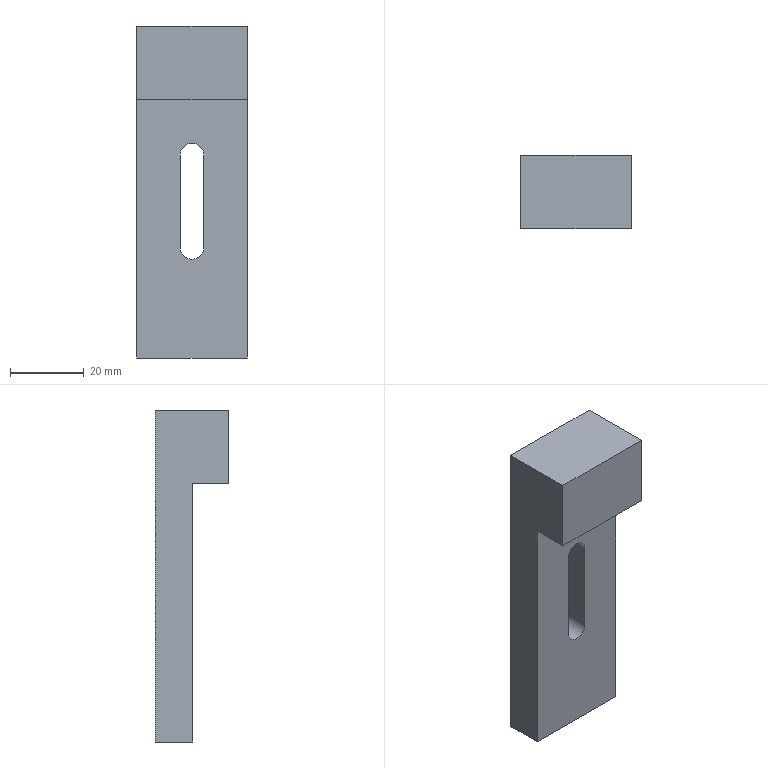Component | SolidWorks | CS021-A10-A012-3 | 1 solid | 12 faces | box 30 x 20 x 90 mm | volume 31424 mm3 | plane 10 | cylinder 2 | commonest cylinder face diameters 6.5 x2 | material AL6061
build123d program:
from build123d import *

# Parameters (mm, degrees)
BOSS_EXTRUDE1_DEPTH = 15
CUT_EXTRUDE1_REACH  = 95.408


with BuildPart() as part:
    # Sketch1 → Boss-Extrude1 (new, symmetric)
    with BuildSketch(Plane.XY):
        Polygon((0, 0), (0, 20), (90, 20), (90, 9.8), (20, 9.8), (20, 0), align=None)
    extrude(amount=BOSS_EXTRUDE1_DEPTH, both=True)

    # Sketch2 → Cut-Extrude1 (cut, up to next)
    with BuildSketch(Plane(origin=(0, 20, 0), x_dir=(1, 0, 0), z_dir=(0, 1, 0)), mode=Mode.PRIVATE) as cut_extrude1_sk1:
        with BuildLine():
            Line((35, 3.25), (60, 3.25))
            ThreePointArc((60, 3.25), (63.25, 0), (60, -3.25))
            Line((60, -3.25), (35, -3.25))
            ThreePointArc((35, -3.25), (31.75, 0), (35, 3.25))
        make_face()
    cut_extrude1_tool1 = extrude(cut_extrude1_sk1.sketch, amount=-CUT_EXTRUDE1_REACH, mode=Mode.PRIVATE) & part.part
    add(cut_extrude1_tool1.solids().sort_by_distance((47.5, 20, 0))[0], mode=Mode.SUBTRACT)


solid = part.part

# Placed as in the assembly
solid = solid.moved(Location((197.949, 15.017, 130), (0, 90, 0)))
STEP:
#1=COLOUR_RGB('',0.7922,0.8196,0.9333);
#2=FILL_AREA_STYLE_COLOUR('',#1);
#3=FILL_AREA_STYLE('',(#2));
#4=SURFACE_STYLE_FILL_AREA(#3);
#5=SURFACE_SIDE_STYLE('',(#4));
#6=SURFACE_STYLE_USAGE(.BOTH.,#5);
#7=PRESENTATION_STYLE_ASSIGNMENT((#6));
#8=CARTESIAN_POINT('',(7.203,0.5912,5.118));
#9=VERTEX_POINT('',#8);
#10=CARTESIAN_POINT('',(7.203,0.5912,4.331));
#11=VERTEX_POINT('',#10);
#12=CARTESIAN_POINT('',(7.203,0.5912,4.331));
#13=DIRECTION('',(0.,-0.,-1.));
#14=VECTOR('',#13,39.37);
#15=LINE('',#12,#14);
#16=EDGE_CURVE('',#9,#11,#15,.T.);
#17=ORIENTED_EDGE('',*,*,#16,.T.);
#18=CARTESIAN_POINT('',(8.384,0.5912,4.331));
#19=VERTEX_POINT('',#18);
#20=CARTESIAN_POINT('',(8.384,0.5912,4.331));
#21=DIRECTION('',(-1.,0.,0.));
#22=VECTOR('',#21,39.37);
#23=LINE('',#20,#22);
#24=EDGE_CURVE('',#19,#11,#23,.T.);
#25=ORIENTED_EDGE('',*,*,#24,.F.);
#26=CARTESIAN_POINT('',(8.384,0.5912,5.118));
#27=VERTEX_POINT('',#26);
#28=CARTESIAN_POINT('',(8.384,0.5912,4.331));
#29=DIRECTION('',(0.,-0.,-1.));
#30=VECTOR('',#29,39.37);
#31=LINE('',#28,#30);
#32=EDGE_CURVE('',#27,#19,#31,.T.);
#33=ORIENTED_EDGE('',*,*,#32,.F.);
#34=CARTESIAN_POINT('',(8.384,0.5912,5.118));
#35=DIRECTION('',(-1.,0.,0.));
#36=VECTOR('',#35,39.37);
#37=LINE('',#34,#36);
#38=EDGE_CURVE('',#27,#9,#37,.T.);
#39=ORIENTED_EDGE('',*,*,#38,.T.);
#40=EDGE_LOOP('',(#17,#25,#33,#39));
#41=FACE_OUTER_BOUND('',#40,.T.);
#42=CARTESIAN_POINT('',(8.384,0.5912,4.331));
#43=DIRECTION('',(0.,1.,-0.));
#44=DIRECTION('',(1.,-0.,0.));
#45=AXIS2_PLACEMENT_3D('',#42,#43,#44);
#46=PLANE('',#45);
#47=ADVANCED_FACE('',(#41),#46,.F.);
#48=CARTESIAN_POINT('',(7.203,0.977,4.331));
#49=VERTEX_POINT('',#48);
#50=CARTESIAN_POINT('',(7.203,0.977,4.331));
#51=DIRECTION('',(0.,1.,-0.));
#52=VECTOR('',#51,39.37);
#53=LINE('',#50,#52);
#54=EDGE_CURVE('',#11,#49,#53,.T.);
#55=ORIENTED_EDGE('',*,*,#54,.T.);
#56=CARTESIAN_POINT('',(8.384,0.977,4.331));
#57=VERTEX_POINT('',#56);
#58=CARTESIAN_POINT('',(8.384,0.977,4.331));
#59=DIRECTION('',(-1.,0.,0.));
#60=VECTOR('',#59,39.37);
#61=LINE('',#58,#60);
#62=EDGE_CURVE('',#57,#49,#61,.T.);
#63=ORIENTED_EDGE('',*,*,#62,.F.);
#64=CARTESIAN_POINT('',(8.384,0.977,4.331));
#65=DIRECTION('',(0.,1.,-0.));
#66=VECTOR('',#65,39.37);
#67=LINE('',#64,#66);
#68=EDGE_CURVE('',#19,#57,#67,.T.);
#69=ORIENTED_EDGE('',*,*,#68,.F.);
#70=ORIENTED_EDGE('',*,*,#24,.T.);
#71=EDGE_LOOP('',(#55,#63,#69,#70));
#72=FACE_OUTER_BOUND('',#71,.T.);
#73=CARTESIAN_POINT('',(8.384,0.977,4.331));
#74=DIRECTION('',(-0.,0.,1.));
#75=DIRECTION('',(-0.,-1.,0.));
#76=AXIS2_PLACEMENT_3D('',#73,#74,#75);
#77=PLANE('',#76);
#78=ADVANCED_FACE('',(#72),#77,.F.);
#79=CARTESIAN_POINT('',(7.665,0.977,3.74));
#80=VERTEX_POINT('',#79);
#81=CARTESIAN_POINT('',(7.665,0.977,2.756));
#82=VERTEX_POINT('',#81);
#83=CARTESIAN_POINT('',(7.665,0.977,3.74));
#84=DIRECTION('',(0.,0.,-1.));
#85=VECTOR('',#84,39.37);
#86=LINE('',#83,#85);
#87=EDGE_CURVE('',#80,#82,#86,.T.);
#88=ORIENTED_EDGE('',*,*,#87,.F.);
#89=CARTESIAN_POINT('',(7.921,0.977,3.74));
#90=VERTEX_POINT('',#89);
#91=CARTESIAN_POINT('',(7.793,0.977,3.74));
#92=DIRECTION('',(-0.,-1.,-0.));
#93=DIRECTION('',(0.,0.,1.));
#94=AXIS2_PLACEMENT_3D('',#91,#92,#93);
#95=CIRCLE('',#94,0.128);
#96=EDGE_CURVE('',#90,#80,#95,.T.);
#97=ORIENTED_EDGE('',*,*,#96,.F.);
#98=CARTESIAN_POINT('',(7.921,0.977,2.756));
#99=VERTEX_POINT('',#98);
#100=CARTESIAN_POINT('',(7.921,0.977,3.74));
#101=DIRECTION('',(-0.,-0.,1.));
#102=VECTOR('',#101,39.37);
#103=LINE('',#100,#102);
#104=EDGE_CURVE('',#99,#90,#103,.T.);
#105=ORIENTED_EDGE('',*,*,#104,.F.);
#106=CARTESIAN_POINT('',(7.793,0.977,2.756));
#107=DIRECTION('',(-0.,-1.,-0.));
#108=DIRECTION('',(0.,0.,1.));
#109=AXIS2_PLACEMENT_3D('',#106,#107,#108);
#110=CIRCLE('',#109,0.128);
#111=EDGE_CURVE('',#82,#99,#110,.T.);
#112=ORIENTED_EDGE('',*,*,#111,.F.);
#113=EDGE_LOOP('',(#88,#97,#105,#112));
#114=FACE_BOUND('',#113,.T.);
#115=CARTESIAN_POINT('',(7.203,0.977,1.575));
#116=VERTEX_POINT('',#115);
#117=CARTESIAN_POINT('',(7.203,0.977,1.575));
#118=DIRECTION('',(0.,0.,-1.));
#119=VECTOR('',#118,39.37);
#120=LINE('',#117,#119);
#121=EDGE_CURVE('',#49,#116,#120,.T.);
#122=ORIENTED_EDGE('',*,*,#121,.T.);
#123=CARTESIAN_POINT('',(8.384,0.977,1.575));
#124=VERTEX_POINT('',#123);
#125=CARTESIAN_POINT('',(8.384,0.977,1.575));
#126=DIRECTION('',(-1.,0.,0.));
#127=VECTOR('',#126,39.37);
#128=LINE('',#125,#127);
#129=EDGE_CURVE('',#124,#116,#128,.T.);
#130=ORIENTED_EDGE('',*,*,#129,.F.);
#131=CARTESIAN_POINT('',(8.384,0.977,1.575));
#132=DIRECTION('',(0.,0.,-1.));
#133=VECTOR('',#132,39.37);
#134=LINE('',#131,#133);
#135=EDGE_CURVE('',#57,#124,#134,.T.);
#136=ORIENTED_EDGE('',*,*,#135,.F.);
#137=ORIENTED_EDGE('',*,*,#62,.T.);
#138=EDGE_LOOP('',(#122,#130,#136,#137));
#139=FACE_OUTER_BOUND('',#138,.T.);
#140=CARTESIAN_POINT('',(8.384,0.977,1.575));
#141=DIRECTION('',(0.,1.,0.));
#142=DIRECTION('',(-0.,-0.,1.));
#143=AXIS2_PLACEMENT_3D('',#140,#141,#142);
#144=PLANE('',#143);
#145=ADVANCED_FACE('',(#114,#139),#144,.F.);
#146=CARTESIAN_POINT('',(7.203,1.379,1.575));
#147=VERTEX_POINT('',#146);
#148=CARTESIAN_POINT('',(7.203,1.379,1.575));
#149=DIRECTION('',(0.,1.,-0.));
#150=VECTOR('',#149,39.37);
#151=LINE('',#148,#150);
#152=EDGE_CURVE('',#116,#147,#151,.T.);
#153=ORIENTED_EDGE('',*,*,#152,.T.);
#154=CARTESIAN_POINT('',(8.384,1.379,1.575));
#155=VERTEX_POINT('',#154);
#156=CARTESIAN_POINT('',(8.384,1.379,1.575));
#157=DIRECTION('',(-1.,0.,0.));
#158=VECTOR('',#157,39.37);
#159=LINE('',#156,#158);
#160=EDGE_CURVE('',#155,#147,#159,.T.);
#161=ORIENTED_EDGE('',*,*,#160,.F.);
#162=CARTESIAN_POINT('',(8.384,1.379,1.575));
#163=DIRECTION('',(0.,1.,-0.));
#164=VECTOR('',#163,39.37);
#165=LINE('',#162,#164);
#166=EDGE_CURVE('',#124,#155,#165,.T.);
#167=ORIENTED_EDGE('',*,*,#166,.F.);
#168=ORIENTED_EDGE('',*,*,#129,.T.);
#169=EDGE_LOOP('',(#153,#161,#167,#168));
#170=FACE_OUTER_BOUND('',#169,.T.);
#171=CARTESIAN_POINT('',(8.384,1.379,1.575));
#172=DIRECTION('',(0.,0.,1.));
#173=DIRECTION('',(1.,-0.,0.));
#174=AXIS2_PLACEMENT_3D('',#171,#172,#173);
#175=PLANE('',#174);
#176=ADVANCED_FACE('',(#170),#175,.F.);
#177=CARTESIAN_POINT('',(7.921,1.379,3.74));
#178=VERTEX_POINT('',#177);
#179=CARTESIAN_POINT('',(7.921,1.379,2.756));
#180=VERTEX_POINT('',#179);
#181=CARTESIAN_POINT('',(7.921,1.379,3.74));
#182=DIRECTION('',(0.,-0.,-1.));
#183=VECTOR('',#182,39.37);
#184=LINE('',#181,#183);
#185=EDGE_CURVE('',#178,#180,#184,.T.);
#186=ORIENTED_EDGE('',*,*,#185,.F.);
#187=CARTESIAN_POINT('',(7.665,1.379,3.74));
#188=VERTEX_POINT('',#187);
#189=CARTESIAN_POINT('',(7.793,1.379,3.74));
#190=DIRECTION('',(0.,1.,-0.));
#191=DIRECTION('',(1.,0.,0.));
#192=AXIS2_PLACEMENT_3D('',#189,#190,#191);
#193=CIRCLE('',#192,0.128);
#194=EDGE_CURVE('',#188,#178,#193,.T.);
#195=ORIENTED_EDGE('',*,*,#194,.F.);
#196=CARTESIAN_POINT('',(7.665,1.379,2.756));
#197=VERTEX_POINT('',#196);
#198=CARTESIAN_POINT('',(7.665,1.379,3.74));
#199=DIRECTION('',(-0.,0.,1.));
#200=VECTOR('',#199,39.37);
#201=LINE('',#198,#200);
#202=EDGE_CURVE('',#197,#188,#201,.T.);
#203=ORIENTED_EDGE('',*,*,#202,.F.);
#204=CARTESIAN_POINT('',(7.793,1.379,2.756));
#205=DIRECTION('',(0.,1.,-0.));
#206=DIRECTION('',(1.,0.,0.));
#207=AXIS2_PLACEMENT_3D('',#204,#205,#206);
#208=CIRCLE('',#207,0.128);
#209=EDGE_CURVE('',#180,#197,#208,.T.);
#210=ORIENTED_EDGE('',*,*,#209,.F.);
#211=EDGE_LOOP('',(#186,#195,#203,#210));
#212=FACE_BOUND('',#211,.T.);
#213=CARTESIAN_POINT('',(7.203,1.379,5.118));
#214=VERTEX_POINT('',#213);
#215=CARTESIAN_POINT('',(7.203,1.379,5.118));
#216=DIRECTION('',(-0.,0.,1.));
#217=VECTOR('',#216,39.37);
#218=LINE('',#215,#217);
#219=EDGE_CURVE('',#147,#214,#218,.T.);
#220=ORIENTED_EDGE('',*,*,#219,.T.);
#221=CARTESIAN_POINT('',(8.384,1.379,5.118));
#222=VERTEX_POINT('',#221);
#223=CARTESIAN_POINT('',(8.384,1.379,5.118));
#224=DIRECTION('',(-1.,0.,0.));
#225=VECTOR('',#224,39.37);
#226=LINE('',#223,#225);
#227=EDGE_CURVE('',#222,#214,#226,.T.);
#228=ORIENTED_EDGE('',*,*,#227,.F.);
#229=CARTESIAN_POINT('',(8.384,1.379,5.118));
#230=DIRECTION('',(-0.,0.,1.));
#231=VECTOR('',#230,39.37);
#232=LINE('',#229,#231);
#233=EDGE_CURVE('',#155,#222,#232,.T.);
#234=ORIENTED_EDGE('',*,*,#233,.F.);
#235=ORIENTED_EDGE('',*,*,#160,.T.);
#236=EDGE_LOOP('',(#220,#228,#234,#235));
#237=FACE_OUTER_BOUND('',#236,.T.);
#238=CARTESIAN_POINT('',(8.384,1.379,5.118));
#239=DIRECTION('',(-0.,-1.,0.));
#240=DIRECTION('',(-1.,0.,0.));
#241=AXIS2_PLACEMENT_3D('',#238,#239,#240);
#242=PLANE('',#241);
#243=ADVANCED_FACE('',(#212,#237),#242,.F.);
#244=CARTESIAN_POINT('',(7.203,0.5912,5.118));
#245=DIRECTION('',(-0.,-1.,0.));
#246=VECTOR('',#245,39.37);
#247=LINE('',#244,#246);
#248=EDGE_CURVE('',#214,#9,#247,.T.);
#249=ORIENTED_EDGE('',*,*,#248,.T.);
#250=ORIENTED_EDGE('',*,*,#38,.F.);
#251=CARTESIAN_POINT('',(8.384,0.5912,5.118));
#252=DIRECTION('',(-0.,-1.,0.));
#253=VECTOR('',#252,39.37);
#254=LINE('',#251,#253);
#255=EDGE_CURVE('',#222,#27,#254,.T.);
#256=ORIENTED_EDGE('',*,*,#255,.F.);
#257=ORIENTED_EDGE('',*,*,#227,.T.);
#258=EDGE_LOOP('',(#249,#250,#256,#257));
#259=FACE_OUTER_BOUND('',#258,.T.);
#260=CARTESIAN_POINT('',(8.384,0.5912,5.118));
#261=DIRECTION('',(-0.,-0.,-1.));
#262=DIRECTION('',(-1.,0.,0.));
#263=AXIS2_PLACEMENT_3D('',#260,#261,#262);
#264=PLANE('',#263);
#265=ADVANCED_FACE('',(#259),#264,.F.);
#266=ORIENTED_EDGE('',*,*,#32,.T.);
#267=ORIENTED_EDGE('',*,*,#68,.T.);
#268=ORIENTED_EDGE('',*,*,#135,.T.);
#269=ORIENTED_EDGE('',*,*,#166,.T.);
#270=ORIENTED_EDGE('',*,*,#233,.T.);
#271=ORIENTED_EDGE('',*,*,#255,.T.);
#272=EDGE_LOOP('',(#266,#267,#268,#269,#270,#271));
#273=FACE_OUTER_BOUND('',#272,.T.);
#274=CARTESIAN_POINT('',(8.384,0.5912,5.118));
#275=DIRECTION('',(-1.,0.,-0.));
#276=DIRECTION('',(-0.,0.,1.));
#277=AXIS2_PLACEMENT_3D('',#274,#275,#276);
#278=PLANE('',#277);
#279=ADVANCED_FACE('',(#273),#278,.F.);
#280=ORIENTED_EDGE('',*,*,#16,.F.);
#281=ORIENTED_EDGE('',*,*,#248,.F.);
#282=ORIENTED_EDGE('',*,*,#219,.F.);
#283=ORIENTED_EDGE('',*,*,#152,.F.);
#284=ORIENTED_EDGE('',*,*,#121,.F.);
#285=ORIENTED_EDGE('',*,*,#54,.F.);
#286=EDGE_LOOP('',(#280,#281,#282,#283,#284,#285));
#287=FACE_OUTER_BOUND('',#286,.T.);
#288=CARTESIAN_POINT('',(7.203,0.5912,5.118));
#289=DIRECTION('',(-1.,0.,-0.));
#290=DIRECTION('',(-0.,0.,1.));
#291=AXIS2_PLACEMENT_3D('',#288,#289,#290);
#292=PLANE('',#291);
#293=ADVANCED_FACE('',(#287),#292,.T.);
#294=ORIENTED_EDGE('',*,*,#96,.T.);
#295=CARTESIAN_POINT('',(7.665,0.5912,3.74));
#296=DIRECTION('',(0.,1.,-0.));
#297=VECTOR('',#296,39.37);
#298=LINE('',#295,#297);
#299=EDGE_CURVE('',#80,#188,#298,.T.);
#300=ORIENTED_EDGE('',*,*,#299,.T.);
#301=ORIENTED_EDGE('',*,*,#194,.T.);
#302=CARTESIAN_POINT('',(7.921,0.5912,3.74));
#303=DIRECTION('',(0.,1.,-0.));
#304=VECTOR('',#303,39.37);
#305=LINE('',#302,#304);
#306=EDGE_CURVE('',#90,#178,#305,.T.);
#307=ORIENTED_EDGE('',*,*,#306,.F.);
#308=EDGE_LOOP('',(#294,#300,#301,#307));
#309=FACE_OUTER_BOUND('',#308,.T.);
#310=CARTESIAN_POINT('',(7.793,0.5912,3.74));
#311=DIRECTION('',(0.,1.,-0.));
#312=DIRECTION('',(1.,0.,0.));
#313=AXIS2_PLACEMENT_3D('',#310,#311,#312);
#314=CYLINDRICAL_SURFACE('',#313,0.128);
#315=ADVANCED_FACE('',(#309),#314,.F.);
#316=ORIENTED_EDGE('',*,*,#87,.T.);
#317=CARTESIAN_POINT('',(7.665,0.5912,2.756));
#318=DIRECTION('',(0.,1.,-0.));
#319=VECTOR('',#318,39.37);
#320=LINE('',#317,#319);
#321=EDGE_CURVE('',#82,#197,#320,.T.);
#322=ORIENTED_EDGE('',*,*,#321,.T.);
#323=ORIENTED_EDGE('',*,*,#202,.T.);
#324=ORIENTED_EDGE('',*,*,#299,.F.);
#325=EDGE_LOOP('',(#316,#322,#323,#324));
#326=FACE_OUTER_BOUND('',#325,.T.);
#327=CARTESIAN_POINT('',(7.665,0.5912,3.74));
#328=DIRECTION('',(-1.,0.,-0.));
#329=DIRECTION('',(-0.,0.,1.));
#330=AXIS2_PLACEMENT_3D('',#327,#328,#329);
#331=PLANE('',#330);
#332=ADVANCED_FACE('',(#326),#331,.F.);
#333=ORIENTED_EDGE('',*,*,#111,.T.);
#334=CARTESIAN_POINT('',(7.921,0.5912,2.756));
#335=DIRECTION('',(0.,1.,-0.));
#336=VECTOR('',#335,39.37);
#337=LINE('',#334,#336);
#338=EDGE_CURVE('',#99,#180,#337,.T.);
#339=ORIENTED_EDGE('',*,*,#338,.T.);
#340=ORIENTED_EDGE('',*,*,#209,.T.);
#341=ORIENTED_EDGE('',*,*,#321,.F.);
#342=EDGE_LOOP('',(#333,#339,#340,#341));
#343=FACE_OUTER_BOUND('',#342,.T.);
#344=CARTESIAN_POINT('',(7.793,0.5912,2.756));
#345=DIRECTION('',(0.,1.,-0.));
#346=DIRECTION('',(1.,0.,0.));
#347=AXIS2_PLACEMENT_3D('',#344,#345,#346);
#348=CYLINDRICAL_SURFACE('',#347,0.128);
#349=ADVANCED_FACE('',(#343),#348,.F.);
#350=ORIENTED_EDGE('',*,*,#104,.T.);
#351=ORIENTED_EDGE('',*,*,#306,.T.);
#352=ORIENTED_EDGE('',*,*,#185,.T.);
#353=ORIENTED_EDGE('',*,*,#338,.F.);
#354=EDGE_LOOP('',(#350,#351,#352,#353));
#355=FACE_OUTER_BOUND('',#354,.T.);
#356=CARTESIAN_POINT('',(7.921,0.5912,3.74));
#357=DIRECTION('',(1.,-0.,0.));
#358=DIRECTION('',(0.,-0.,-1.));
#359=AXIS2_PLACEMENT_3D('',#356,#357,#358);
#360=PLANE('',#359);
#361=ADVANCED_FACE('',(#355),#360,.F.);
#362=CLOSED_SHELL('',(#47,#78,#145,#176,#243,#265,#279,#293,#315,#332,#349,#361));
#363=MANIFOLD_SOLID_BREP('',#362);
#364=STYLED_ITEM('',(#7),#363);
#365=(LENGTH_UNIT()NAMED_UNIT(*)SI_UNIT($,.METRE.));
#366=LENGTH_MEASURE_WITH_UNIT(LENGTH_MEASURE(0.0254),#365);
#367=DIMENSIONAL_EXPONENTS(1.,0.,0.,0.,0.,0.,0.);
#368=(CONVERSION_BASED_UNIT('',#366)LENGTH_UNIT()NAMED_UNIT(#367));
#369=UNCERTAINTY_MEASURE_WITH_UNIT(LENGTH_MEASURE(0.00001),#368,'','');
#370=(NAMED_UNIT(*)PLANE_ANGLE_UNIT()SI_UNIT($,.RADIAN.));
#371=(NAMED_UNIT(*)SI_UNIT($,.STERADIAN.)SOLID_ANGLE_UNIT());
#372=(GEOMETRIC_REPRESENTATION_CONTEXT(3)GLOBAL_UNCERTAINTY_ASSIGNED_CONTEXT((#369))GLOBAL_UNIT_ASSIGNED_CONTEXT((#368,#370,#371))REPRESENTATION_CONTEXT('',''));
#373=MECHANICAL_DESIGN_GEOMETRIC_PRESENTATION_REPRESENTATION('',(#364),#372);
#374=CARTESIAN_POINT('',(0.,0.,0.));
#375=DIRECTION('',(0.,0.,1.));
#376=DIRECTION('',(1.,0.,0.));
#377=AXIS2_PLACEMENT_3D('',#374,#375,#376);
#378=(LENGTH_UNIT()NAMED_UNIT(*)SI_UNIT($,.METRE.));
#379=LENGTH_MEASURE_WITH_UNIT(LENGTH_MEASURE(0.0254),#378);
#380=DIMENSIONAL_EXPONENTS(1.,0.,0.,0.,0.,0.,0.);
#381=(CONVERSION_BASED_UNIT('',#379)LENGTH_UNIT()NAMED_UNIT(#380));
#382=UNCERTAINTY_MEASURE_WITH_UNIT(LENGTH_MEASURE(0.00001),#381,'','');
#383=(NAMED_UNIT(*)PLANE_ANGLE_UNIT()SI_UNIT($,.RADIAN.));
#384=(NAMED_UNIT(*)SI_UNIT($,.STERADIAN.)SOLID_ANGLE_UNIT());
#385=(GEOMETRIC_REPRESENTATION_CONTEXT(3)GLOBAL_UNCERTAINTY_ASSIGNED_CONTEXT((#382))GLOBAL_UNIT_ASSIGNED_CONTEXT((#381,#383,#384))REPRESENTATION_CONTEXT('',''));
#386=ADVANCED_BREP_SHAPE_REPRESENTATION('',(#363,#377),#385);
#387=PRESENTATION_LAYER_ASSIGNMENT('','',(#364));